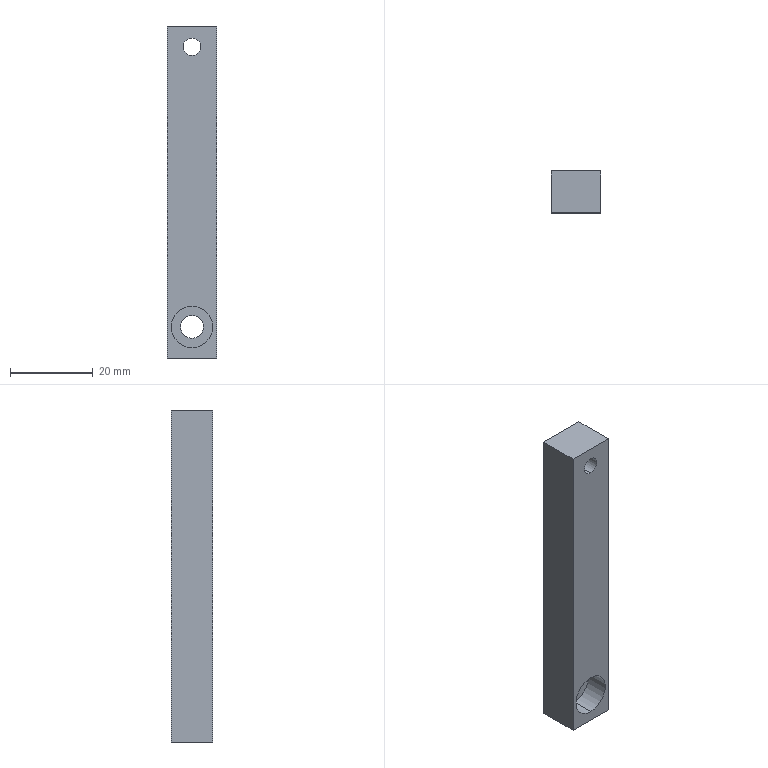Component | SolidWorks | LeftLocatingPlate-1 | 1 solid | 13 faces | box 12 x 10 x 80 mm | volume 8912 mm3 | plane 7 | cylinder 6 | commonest cylinder face diameters 4.2 x2 10 x2 5.5 x2
build123d program:
from build123d import *

# Parameters (mm, degrees)
SKETCH1_W                                         = 80
SKETCH1_H                                         = 12
BOSS_EXTRUDE1_DEPTH                               = 10
HOLE_SIZE_ACCORDING_TO_HEXAGON_SOCKET_D           = 5.5
HOLE_SIZE_ACCORDING_TO_HEXAGON_SOCKET_DEPTH       = 12.4
HOLE_SIZE_ACCORDING_TO_HEXAGON_SOCKET_CBORE_D     = 10
HOLE_SIZE_ACCORDING_TO_HEXAGON_SOCKET_CBORE_DEPTH = 5.7
HOLE_SIZE_ACCORDING_TO_HEXAGON_SOCKET_TIP         = 1.652
M5_TAPPED_HOLE1_D                                 = 4.2


with BuildPart() as part:
    # Sketch1 → Boss-Extrude1 (new body)
    with BuildSketch(Plane.XY):
        with Locations((40, 6)):
            Rectangle(SKETCH1_W, SKETCH1_H)
    extrude(amount=BOSS_EXTRUDE1_DEPTH)

    # Hole Size _According to_ Hexagon Socket
    with Locations(Plane(origin=(72.5, 6, 10), x_dir=(1, 0, 0), z_dir=(0, 0, 1))):
        with Locations((0, 0)):
            CounterBoreHole(HOLE_SIZE_ACCORDING_TO_HEXAGON_SOCKET_D / 2, HOLE_SIZE_ACCORDING_TO_HEXAGON_SOCKET_CBORE_D / 2, HOLE_SIZE_ACCORDING_TO_HEXAGON_SOCKET_CBORE_DEPTH, depth=HOLE_SIZE_ACCORDING_TO_HEXAGON_SOCKET_DEPTH)
            with Locations((0, 0, -(HOLE_SIZE_ACCORDING_TO_HEXAGON_SOCKET_DEPTH + HOLE_SIZE_ACCORDING_TO_HEXAGON_SOCKET_TIP / 2))):  # 118° drill point
                Cone(0, HOLE_SIZE_ACCORDING_TO_HEXAGON_SOCKET_D / 2, HOLE_SIZE_ACCORDING_TO_HEXAGON_SOCKET_TIP, mode=Mode.SUBTRACT)

    # M5 Tapped Hole1 (through all)
    with Locations(Plane(origin=(5, 6, 10), x_dir=(1, 0, 0), z_dir=(0, 0, 1))):
        with Locations((0, 0)):
            Hole(M5_TAPPED_HOLE1_D / 2)


solid = part.part

# Placed as in the assembly
solid = solid.moved(Location((134, -227.728, 136), (90, 0, -90)))
STEP:
#1=COLOUR_RGB('',0.7922,0.8196,0.9333);
#2=FILL_AREA_STYLE_COLOUR('',#1);
#3=FILL_AREA_STYLE('',(#2));
#4=SURFACE_STYLE_FILL_AREA(#3);
#5=SURFACE_SIDE_STYLE('',(#4));
#6=SURFACE_STYLE_USAGE(.BOTH.,#5);
#7=PRESENTATION_STYLE_ASSIGNMENT((#6));
#8=CARTESIAN_POINT('',(5.512,-8.966,5.075));
#9=VERTEX_POINT('',#8);
#10=CARTESIAN_POINT('',(5.512,-8.966,5.24));
#11=VERTEX_POINT('',#10);
#12=CARTESIAN_POINT('',(5.512,-8.966,5.157));
#13=DIRECTION('',(0.,1.,0.));
#14=DIRECTION('',(0.,0.,1.));
#15=AXIS2_PLACEMENT_3D('',#12,#13,#14);
#16=CIRCLE('',#15,0.08268);
#17=EDGE_CURVE('',#9,#11,#16,.T.);
#18=ORIENTED_EDGE('',*,*,#17,.T.);
#19=CARTESIAN_POINT('',(5.512,-9.359,5.24));
#20=VERTEX_POINT('',#19);
#21=CARTESIAN_POINT('',(5.512,-9.359,5.24));
#22=DIRECTION('',(-0.,-1.,-0.));
#23=VECTOR('',#22,39.37);
#24=LINE('',#21,#23);
#25=EDGE_CURVE('',#11,#20,#24,.T.);
#26=ORIENTED_EDGE('',*,*,#25,.T.);
#27=CARTESIAN_POINT('',(5.512,-9.359,5.075));
#28=VERTEX_POINT('',#27);
#29=CARTESIAN_POINT('',(5.512,-9.359,5.157));
#30=DIRECTION('',(-0.,-1.,-0.));
#31=DIRECTION('',(0.,0.,-1.));
#32=AXIS2_PLACEMENT_3D('',#29,#30,#31);
#33=CIRCLE('',#32,0.08268);
#34=EDGE_CURVE('',#20,#28,#33,.T.);
#35=ORIENTED_EDGE('',*,*,#34,.T.);
#36=CARTESIAN_POINT('',(5.512,-9.359,5.075));
#37=DIRECTION('',(-0.,-1.,-0.));
#38=VECTOR('',#37,39.37);
#39=LINE('',#36,#38);
#40=EDGE_CURVE('',#9,#28,#39,.T.);
#41=ORIENTED_EDGE('',*,*,#40,.F.);
#42=EDGE_LOOP('',(#18,#26,#35,#41));
#43=FACE_OUTER_BOUND('',#42,.T.);
#44=CARTESIAN_POINT('',(5.512,-9.359,5.157));
#45=DIRECTION('',(-0.,-1.,-0.));
#46=DIRECTION('',(0.,0.,-1.));
#47=AXIS2_PLACEMENT_3D('',#44,#45,#46);
#48=CYLINDRICAL_SURFACE('',#47,0.08268);
#49=ADVANCED_FACE('',(#43),#48,.F.);
#50=CARTESIAN_POINT('',(5.512,-9.135,2.697));
#51=VERTEX_POINT('',#50);
#52=CARTESIAN_POINT('',(5.512,-9.135,2.303));
#53=VERTEX_POINT('',#52);
#54=CARTESIAN_POINT('',(5.512,-9.135,2.5));
#55=DIRECTION('',(-0.,-1.,-0.));
#56=DIRECTION('',(0.,0.,-1.));
#57=AXIS2_PLACEMENT_3D('',#54,#55,#56);
#58=CIRCLE('',#57,0.1969);
#59=EDGE_CURVE('',#51,#53,#58,.T.);
#60=ORIENTED_EDGE('',*,*,#59,.F.);
#61=CARTESIAN_POINT('',(5.512,-9.359,2.697));
#62=VERTEX_POINT('',#61);
#63=CARTESIAN_POINT('',(5.512,-9.359,2.697));
#64=DIRECTION('',(-0.,-1.,-0.));
#65=VECTOR('',#64,39.37);
#66=LINE('',#63,#65);
#67=EDGE_CURVE('',#51,#62,#66,.T.);
#68=ORIENTED_EDGE('',*,*,#67,.T.);
#69=CARTESIAN_POINT('',(5.512,-9.359,2.303));
#70=VERTEX_POINT('',#69);
#71=CARTESIAN_POINT('',(5.512,-9.359,2.5));
#72=DIRECTION('',(-0.,-1.,-0.));
#73=DIRECTION('',(0.,0.,-1.));
#74=AXIS2_PLACEMENT_3D('',#71,#72,#73);
#75=CIRCLE('',#74,0.1969);
#76=EDGE_CURVE('',#62,#70,#75,.T.);
#77=ORIENTED_EDGE('',*,*,#76,.T.);
#78=CARTESIAN_POINT('',(5.512,-9.359,2.303));
#79=DIRECTION('',(-0.,-1.,-0.));
#80=VECTOR('',#79,39.37);
#81=LINE('',#78,#80);
#82=EDGE_CURVE('',#53,#70,#81,.T.);
#83=ORIENTED_EDGE('',*,*,#82,.F.);
#84=EDGE_LOOP('',(#60,#68,#77,#83));
#85=FACE_OUTER_BOUND('',#84,.T.);
#86=CARTESIAN_POINT('',(5.512,-9.359,2.5));
#87=DIRECTION('',(-0.,-1.,-0.));
#88=DIRECTION('',(0.,0.,-1.));
#89=AXIS2_PLACEMENT_3D('',#86,#87,#88);
#90=CYLINDRICAL_SURFACE('',#89,0.1969);
#91=ADVANCED_FACE('',(#85),#90,.F.);
#92=CARTESIAN_POINT('',(5.512,-8.966,2.392));
#93=VERTEX_POINT('',#92);
#94=CARTESIAN_POINT('',(5.512,-8.966,2.608));
#95=VERTEX_POINT('',#94);
#96=CARTESIAN_POINT('',(5.512,-8.966,2.5));
#97=DIRECTION('',(0.,1.,0.));
#98=DIRECTION('',(0.,0.,1.));
#99=AXIS2_PLACEMENT_3D('',#96,#97,#98);
#100=CIRCLE('',#99,0.1083);
#101=EDGE_CURVE('',#93,#95,#100,.T.);
#102=ORIENTED_EDGE('',*,*,#101,.T.);
#103=CARTESIAN_POINT('',(5.512,-9.135,2.608));
#104=VERTEX_POINT('',#103);
#105=CARTESIAN_POINT('',(5.512,-9.359,2.608));
#106=DIRECTION('',(-0.,-1.,-0.));
#107=VECTOR('',#106,39.37);
#108=LINE('',#105,#107);
#109=EDGE_CURVE('',#95,#104,#108,.T.);
#110=ORIENTED_EDGE('',*,*,#109,.T.);
#111=CARTESIAN_POINT('',(5.512,-9.135,2.392));
#112=VERTEX_POINT('',#111);
#113=CARTESIAN_POINT('',(5.512,-9.135,2.5));
#114=DIRECTION('',(-0.,-1.,-0.));
#115=DIRECTION('',(0.,0.,-1.));
#116=AXIS2_PLACEMENT_3D('',#113,#114,#115);
#117=CIRCLE('',#116,0.1083);
#118=EDGE_CURVE('',#104,#112,#117,.T.);
#119=ORIENTED_EDGE('',*,*,#118,.T.);
#120=CARTESIAN_POINT('',(5.512,-9.359,2.392));
#121=DIRECTION('',(-0.,-1.,-0.));
#122=VECTOR('',#121,39.37);
#123=LINE('',#120,#122);
#124=EDGE_CURVE('',#93,#112,#123,.T.);
#125=ORIENTED_EDGE('',*,*,#124,.F.);
#126=EDGE_LOOP('',(#102,#110,#119,#125));
#127=FACE_OUTER_BOUND('',#126,.T.);
#128=CARTESIAN_POINT('',(5.512,-9.359,2.5));
#129=DIRECTION('',(-0.,-1.,-0.));
#130=DIRECTION('',(0.,0.,-1.));
#131=AXIS2_PLACEMENT_3D('',#128,#129,#130);
#132=CYLINDRICAL_SURFACE('',#131,0.1083);
#133=ADVANCED_FACE('',(#127),#132,.F.);
#134=CARTESIAN_POINT('',(5.748,-8.966,5.354));
#135=VERTEX_POINT('',#134);
#136=CARTESIAN_POINT('',(5.276,-8.966,5.354));
#137=VERTEX_POINT('',#136);
#138=CARTESIAN_POINT('',(5.276,-8.966,5.354));
#139=DIRECTION('',(-1.,0.,-0.));
#140=VECTOR('',#139,39.37);
#141=LINE('',#138,#140);
#142=EDGE_CURVE('',#135,#137,#141,.T.);
#143=ORIENTED_EDGE('',*,*,#142,.T.);
#144=CARTESIAN_POINT('',(5.276,-9.359,5.354));
#145=VERTEX_POINT('',#144);
#146=CARTESIAN_POINT('',(5.276,-9.359,5.354));
#147=DIRECTION('',(0.,1.,0.));
#148=VECTOR('',#147,39.37);
#149=LINE('',#146,#148);
#150=EDGE_CURVE('',#145,#137,#149,.T.);
#151=ORIENTED_EDGE('',*,*,#150,.F.);
#152=CARTESIAN_POINT('',(5.748,-9.359,5.354));
#153=VERTEX_POINT('',#152);
#154=CARTESIAN_POINT('',(5.276,-9.359,5.354));
#155=DIRECTION('',(-1.,0.,-0.));
#156=VECTOR('',#155,39.37);
#157=LINE('',#154,#156);
#158=EDGE_CURVE('',#153,#145,#157,.T.);
#159=ORIENTED_EDGE('',*,*,#158,.F.);
#160=CARTESIAN_POINT('',(5.748,-9.359,5.354));
#161=DIRECTION('',(0.,1.,0.));
#162=VECTOR('',#161,39.37);
#163=LINE('',#160,#162);
#164=EDGE_CURVE('',#153,#135,#163,.T.);
#165=ORIENTED_EDGE('',*,*,#164,.T.);
#166=EDGE_LOOP('',(#143,#151,#159,#165));
#167=FACE_OUTER_BOUND('',#166,.T.);
#168=CARTESIAN_POINT('',(5.276,-9.359,5.354));
#169=DIRECTION('',(0.,0.,-1.));
#170=DIRECTION('',(0.,1.,0.));
#171=AXIS2_PLACEMENT_3D('',#168,#169,#170);
#172=PLANE('',#171);
#173=ADVANCED_FACE('',(#167),#172,.F.);
#174=CARTESIAN_POINT('',(5.276,-8.966,2.205));
#175=VERTEX_POINT('',#174);
#176=CARTESIAN_POINT('',(5.276,-8.966,5.354));
#177=DIRECTION('',(0.,0.,-1.));
#178=VECTOR('',#177,39.37);
#179=LINE('',#176,#178);
#180=EDGE_CURVE('',#137,#175,#179,.T.);
#181=ORIENTED_EDGE('',*,*,#180,.T.);
#182=CARTESIAN_POINT('',(5.276,-9.359,2.205));
#183=VERTEX_POINT('',#182);
#184=CARTESIAN_POINT('',(5.276,-9.359,2.205));
#185=DIRECTION('',(0.,1.,0.));
#186=VECTOR('',#185,39.37);
#187=LINE('',#184,#186);
#188=EDGE_CURVE('',#183,#175,#187,.T.);
#189=ORIENTED_EDGE('',*,*,#188,.F.);
#190=CARTESIAN_POINT('',(5.276,-9.359,5.354));
#191=DIRECTION('',(0.,0.,-1.));
#192=VECTOR('',#191,39.37);
#193=LINE('',#190,#192);
#194=EDGE_CURVE('',#145,#183,#193,.T.);
#195=ORIENTED_EDGE('',*,*,#194,.F.);
#196=ORIENTED_EDGE('',*,*,#150,.T.);
#197=EDGE_LOOP('',(#181,#189,#195,#196));
#198=FACE_OUTER_BOUND('',#197,.T.);
#199=CARTESIAN_POINT('',(5.276,-9.359,5.354));
#200=DIRECTION('',(1.,-0.,0.));
#201=DIRECTION('',(-0.,-1.,-0.));
#202=AXIS2_PLACEMENT_3D('',#199,#200,#201);
#203=PLANE('',#202);
#204=ADVANCED_FACE('',(#198),#203,.F.);
#205=CARTESIAN_POINT('',(5.748,-8.966,2.205));
#206=VERTEX_POINT('',#205);
#207=CARTESIAN_POINT('',(5.276,-8.966,2.205));
#208=DIRECTION('',(1.,-0.,0.));
#209=VECTOR('',#208,39.37);
#210=LINE('',#207,#209);
#211=EDGE_CURVE('',#175,#206,#210,.T.);
#212=ORIENTED_EDGE('',*,*,#211,.T.);
#213=CARTESIAN_POINT('',(5.748,-9.359,2.205));
#214=VERTEX_POINT('',#213);
#215=CARTESIAN_POINT('',(5.748,-9.359,2.205));
#216=DIRECTION('',(0.,1.,0.));
#217=VECTOR('',#216,39.37);
#218=LINE('',#215,#217);
#219=EDGE_CURVE('',#214,#206,#218,.T.);
#220=ORIENTED_EDGE('',*,*,#219,.F.);
#221=CARTESIAN_POINT('',(5.276,-9.359,2.205));
#222=DIRECTION('',(1.,-0.,0.));
#223=VECTOR('',#222,39.37);
#224=LINE('',#221,#223);
#225=EDGE_CURVE('',#183,#214,#224,.T.);
#226=ORIENTED_EDGE('',*,*,#225,.F.);
#227=ORIENTED_EDGE('',*,*,#188,.T.);
#228=EDGE_LOOP('',(#212,#220,#226,#227));
#229=FACE_OUTER_BOUND('',#228,.T.);
#230=CARTESIAN_POINT('',(5.276,-9.359,2.205));
#231=DIRECTION('',(-0.,-0.,1.));
#232=DIRECTION('',(-0.,-1.,-0.));
#233=AXIS2_PLACEMENT_3D('',#230,#231,#232);
#234=PLANE('',#233);
#235=ADVANCED_FACE('',(#229),#234,.F.);
#236=CARTESIAN_POINT('',(5.748,-8.966,5.354));
#237=DIRECTION('',(-0.,-0.,1.));
#238=VECTOR('',#237,39.37);
#239=LINE('',#236,#238);
#240=EDGE_CURVE('',#206,#135,#239,.T.);
#241=ORIENTED_EDGE('',*,*,#240,.T.);
#242=ORIENTED_EDGE('',*,*,#164,.F.);
#243=CARTESIAN_POINT('',(5.748,-9.359,5.354));
#244=DIRECTION('',(-0.,-0.,1.));
#245=VECTOR('',#244,39.37);
#246=LINE('',#243,#245);
#247=EDGE_CURVE('',#214,#153,#246,.T.);
#248=ORIENTED_EDGE('',*,*,#247,.F.);
#249=ORIENTED_EDGE('',*,*,#219,.T.);
#250=EDGE_LOOP('',(#241,#242,#248,#249));
#251=FACE_OUTER_BOUND('',#250,.T.);
#252=CARTESIAN_POINT('',(5.748,-9.359,5.354));
#253=DIRECTION('',(-1.,0.,-0.));
#254=DIRECTION('',(0.,1.,0.));
#255=AXIS2_PLACEMENT_3D('',#252,#253,#254);
#256=PLANE('',#255);
#257=ADVANCED_FACE('',(#251),#256,.F.);
#258=CARTESIAN_POINT('',(5.512,-9.359,5.157));
#259=DIRECTION('',(-0.,-1.,-0.));
#260=DIRECTION('',(0.,0.,-1.));
#261=AXIS2_PLACEMENT_3D('',#258,#259,#260);
#262=CIRCLE('',#261,0.08268);
#263=EDGE_CURVE('',#28,#20,#262,.T.);
#264=ORIENTED_EDGE('',*,*,#263,.F.);
#265=ORIENTED_EDGE('',*,*,#34,.F.);
#266=EDGE_LOOP('',(#264,#265));
#267=FACE_BOUND('',#266,.T.);
#268=CARTESIAN_POINT('',(5.512,-9.359,2.5));
#269=DIRECTION('',(-0.,-1.,-0.));
#270=DIRECTION('',(0.,0.,-1.));
#271=AXIS2_PLACEMENT_3D('',#268,#269,#270);
#272=CIRCLE('',#271,0.1969);
#273=EDGE_CURVE('',#70,#62,#272,.T.);
#274=ORIENTED_EDGE('',*,*,#273,.F.);
#275=ORIENTED_EDGE('',*,*,#76,.F.);
#276=EDGE_LOOP('',(#274,#275));
#277=FACE_BOUND('',#276,.T.);
#278=ORIENTED_EDGE('',*,*,#158,.T.);
#279=ORIENTED_EDGE('',*,*,#194,.T.);
#280=ORIENTED_EDGE('',*,*,#225,.T.);
#281=ORIENTED_EDGE('',*,*,#247,.T.);
#282=EDGE_LOOP('',(#278,#279,#280,#281));
#283=FACE_OUTER_BOUND('',#282,.T.);
#284=CARTESIAN_POINT('',(5.276,-9.359,5.354));
#285=DIRECTION('',(0.,1.,0.));
#286=DIRECTION('',(-0.,-0.,1.));
#287=AXIS2_PLACEMENT_3D('',#284,#285,#286);
#288=PLANE('',#287);
#289=ADVANCED_FACE('',(#267,#277,#283),#288,.F.);
#290=ORIENTED_EDGE('',*,*,#17,.F.);
#291=CARTESIAN_POINT('',(5.512,-8.966,5.157));
#292=DIRECTION('',(0.,1.,0.));
#293=DIRECTION('',(0.,0.,1.));
#294=AXIS2_PLACEMENT_3D('',#291,#292,#293);
#295=CIRCLE('',#294,0.08268);
#296=EDGE_CURVE('',#11,#9,#295,.T.);
#297=ORIENTED_EDGE('',*,*,#296,.F.);
#298=EDGE_LOOP('',(#290,#297));
#299=FACE_BOUND('',#298,.T.);
#300=ORIENTED_EDGE('',*,*,#101,.F.);
#301=CARTESIAN_POINT('',(5.512,-8.966,2.5));
#302=DIRECTION('',(0.,1.,0.));
#303=DIRECTION('',(0.,0.,1.));
#304=AXIS2_PLACEMENT_3D('',#301,#302,#303);
#305=CIRCLE('',#304,0.1083);
#306=EDGE_CURVE('',#95,#93,#305,.T.);
#307=ORIENTED_EDGE('',*,*,#306,.F.);
#308=EDGE_LOOP('',(#300,#307));
#309=FACE_BOUND('',#308,.T.);
#310=ORIENTED_EDGE('',*,*,#142,.F.);
#311=ORIENTED_EDGE('',*,*,#240,.F.);
#312=ORIENTED_EDGE('',*,*,#211,.F.);
#313=ORIENTED_EDGE('',*,*,#180,.F.);
#314=EDGE_LOOP('',(#310,#311,#312,#313));
#315=FACE_OUTER_BOUND('',#314,.T.);
#316=CARTESIAN_POINT('',(5.276,-8.966,5.354));
#317=DIRECTION('',(0.,1.,0.));
#318=DIRECTION('',(-0.,-0.,1.));
#319=AXIS2_PLACEMENT_3D('',#316,#317,#318);
#320=PLANE('',#319);
#321=ADVANCED_FACE('',(#299,#309,#315),#320,.T.);
#322=ORIENTED_EDGE('',*,*,#109,.F.);
#323=ORIENTED_EDGE('',*,*,#306,.T.);
#324=ORIENTED_EDGE('',*,*,#124,.T.);
#325=CARTESIAN_POINT('',(5.512,-9.135,2.5));
#326=DIRECTION('',(-0.,-1.,-0.));
#327=DIRECTION('',(0.,0.,-1.));
#328=AXIS2_PLACEMENT_3D('',#325,#326,#327);
#329=CIRCLE('',#328,0.1083);
#330=EDGE_CURVE('',#112,#104,#329,.T.);
#331=ORIENTED_EDGE('',*,*,#330,.T.);
#332=EDGE_LOOP('',(#322,#323,#324,#331));
#333=FACE_OUTER_BOUND('',#332,.T.);
#334=CARTESIAN_POINT('',(5.512,-9.359,2.5));
#335=DIRECTION('',(-0.,-1.,-0.));
#336=DIRECTION('',(0.,0.,-1.));
#337=AXIS2_PLACEMENT_3D('',#334,#335,#336);
#338=CYLINDRICAL_SURFACE('',#337,0.1083);
#339=ADVANCED_FACE('',(#333),#338,.F.);
#340=ORIENTED_EDGE('',*,*,#330,.F.);
#341=ORIENTED_EDGE('',*,*,#118,.F.);
#342=EDGE_LOOP('',(#340,#341));
#343=FACE_BOUND('',#342,.T.);
#344=CARTESIAN_POINT('',(5.512,-9.135,2.5));
#345=DIRECTION('',(-0.,-1.,-0.));
#346=DIRECTION('',(0.,0.,-1.));
#347=AXIS2_PLACEMENT_3D('',#344,#345,#346);
#348=CIRCLE('',#347,0.1969);
#349=EDGE_CURVE('',#53,#51,#348,.T.);
#350=ORIENTED_EDGE('',*,*,#349,.T.);
#351=ORIENTED_EDGE('',*,*,#59,.T.);
#352=EDGE_LOOP('',(#350,#351));
#353=FACE_OUTER_BOUND('',#352,.T.);
#354=CARTESIAN_POINT('',(5.512,-9.135,2.392));
#355=DIRECTION('',(0.,1.,0.));
#356=DIRECTION('',(-0.,-0.,1.));
#357=AXIS2_PLACEMENT_3D('',#354,#355,#356);
#358=PLANE('',#357);
#359=ADVANCED_FACE('',(#343,#353),#358,.F.);
#360=ORIENTED_EDGE('',*,*,#67,.F.);
#361=ORIENTED_EDGE('',*,*,#349,.F.);
#362=ORIENTED_EDGE('',*,*,#82,.T.);
#363=ORIENTED_EDGE('',*,*,#273,.T.);
#364=EDGE_LOOP('',(#360,#361,#362,#363));
#365=FACE_OUTER_BOUND('',#364,.T.);
#366=CARTESIAN_POINT('',(5.512,-9.359,2.5));
#367=DIRECTION('',(-0.,-1.,-0.));
#368=DIRECTION('',(0.,0.,-1.));
#369=AXIS2_PLACEMENT_3D('',#366,#367,#368);
#370=CYLINDRICAL_SURFACE('',#369,0.1969);
#371=ADVANCED_FACE('',(#365),#370,.F.);
#372=ORIENTED_EDGE('',*,*,#25,.F.);
#373=ORIENTED_EDGE('',*,*,#296,.T.);
#374=ORIENTED_EDGE('',*,*,#40,.T.);
#375=ORIENTED_EDGE('',*,*,#263,.T.);
#376=EDGE_LOOP('',(#372,#373,#374,#375));
#377=FACE_OUTER_BOUND('',#376,.T.);
#378=CARTESIAN_POINT('',(5.512,-9.359,5.157));
#379=DIRECTION('',(-0.,-1.,-0.));
#380=DIRECTION('',(0.,0.,-1.));
#381=AXIS2_PLACEMENT_3D('',#378,#379,#380);
#382=CYLINDRICAL_SURFACE('',#381,0.08268);
#383=ADVANCED_FACE('',(#377),#382,.F.);
#384=CLOSED_SHELL('',(#49,#91,#133,#173,#204,#235,#257,#289,#321,#339,#359,#371,#383));
#385=MANIFOLD_SOLID_BREP('',#384);
#386=STYLED_ITEM('',(#7),#385);
#387=(LENGTH_UNIT()NAMED_UNIT(*)SI_UNIT($,.METRE.));
#388=LENGTH_MEASURE_WITH_UNIT(LENGTH_MEASURE(0.0254),#387);
#389=DIMENSIONAL_EXPONENTS(1.,0.,0.,0.,0.,0.,0.);
#390=(CONVERSION_BASED_UNIT('',#388)LENGTH_UNIT()NAMED_UNIT(#389));
#391=UNCERTAINTY_MEASURE_WITH_UNIT(LENGTH_MEASURE(0.00001),#390,'','');
#392=(NAMED_UNIT(*)PLANE_ANGLE_UNIT()SI_UNIT($,.RADIAN.));
#393=(NAMED_UNIT(*)SI_UNIT($,.STERADIAN.)SOLID_ANGLE_UNIT());
#394=(GEOMETRIC_REPRESENTATION_CONTEXT(3)GLOBAL_UNCERTAINTY_ASSIGNED_CONTEXT((#391))GLOBAL_UNIT_ASSIGNED_CONTEXT((#390,#392,#393))REPRESENTATION_CONTEXT('',''));
#395=MECHANICAL_DESIGN_GEOMETRIC_PRESENTATION_REPRESENTATION('',(#386),#394);
#396=PRESENTATION_LAYER_ASSIGNMENT('','',(#386));
#397=CARTESIAN_POINT('',(0.,0.,0.));
#398=DIRECTION('',(0.,0.,1.));
#399=DIRECTION('',(1.,0.,0.));
#400=AXIS2_PLACEMENT_3D('',#397,#398,#399);
#401=(LENGTH_UNIT()NAMED_UNIT(*)SI_UNIT($,.METRE.));
#402=LENGTH_MEASURE_WITH_UNIT(LENGTH_MEASURE(0.0254),#401);
#403=DIMENSIONAL_EXPONENTS(1.,0.,0.,0.,0.,0.,0.);
#404=(CONVERSION_BASED_UNIT('',#402)LENGTH_UNIT()NAMED_UNIT(#403));
#405=UNCERTAINTY_MEASURE_WITH_UNIT(LENGTH_MEASURE(0.00001),#404,'','');
#406=(NAMED_UNIT(*)PLANE_ANGLE_UNIT()SI_UNIT($,.RADIAN.));
#407=(NAMED_UNIT(*)SI_UNIT($,.STERADIAN.)SOLID_ANGLE_UNIT());
#408=(GEOMETRIC_REPRESENTATION_CONTEXT(3)GLOBAL_UNCERTAINTY_ASSIGNED_CONTEXT((#405))GLOBAL_UNIT_ASSIGNED_CONTEXT((#404,#406,#407))REPRESENTATION_CONTEXT('',''));
#409=ADVANCED_BREP_SHAPE_REPRESENTATION('',(#385,#400),#408);